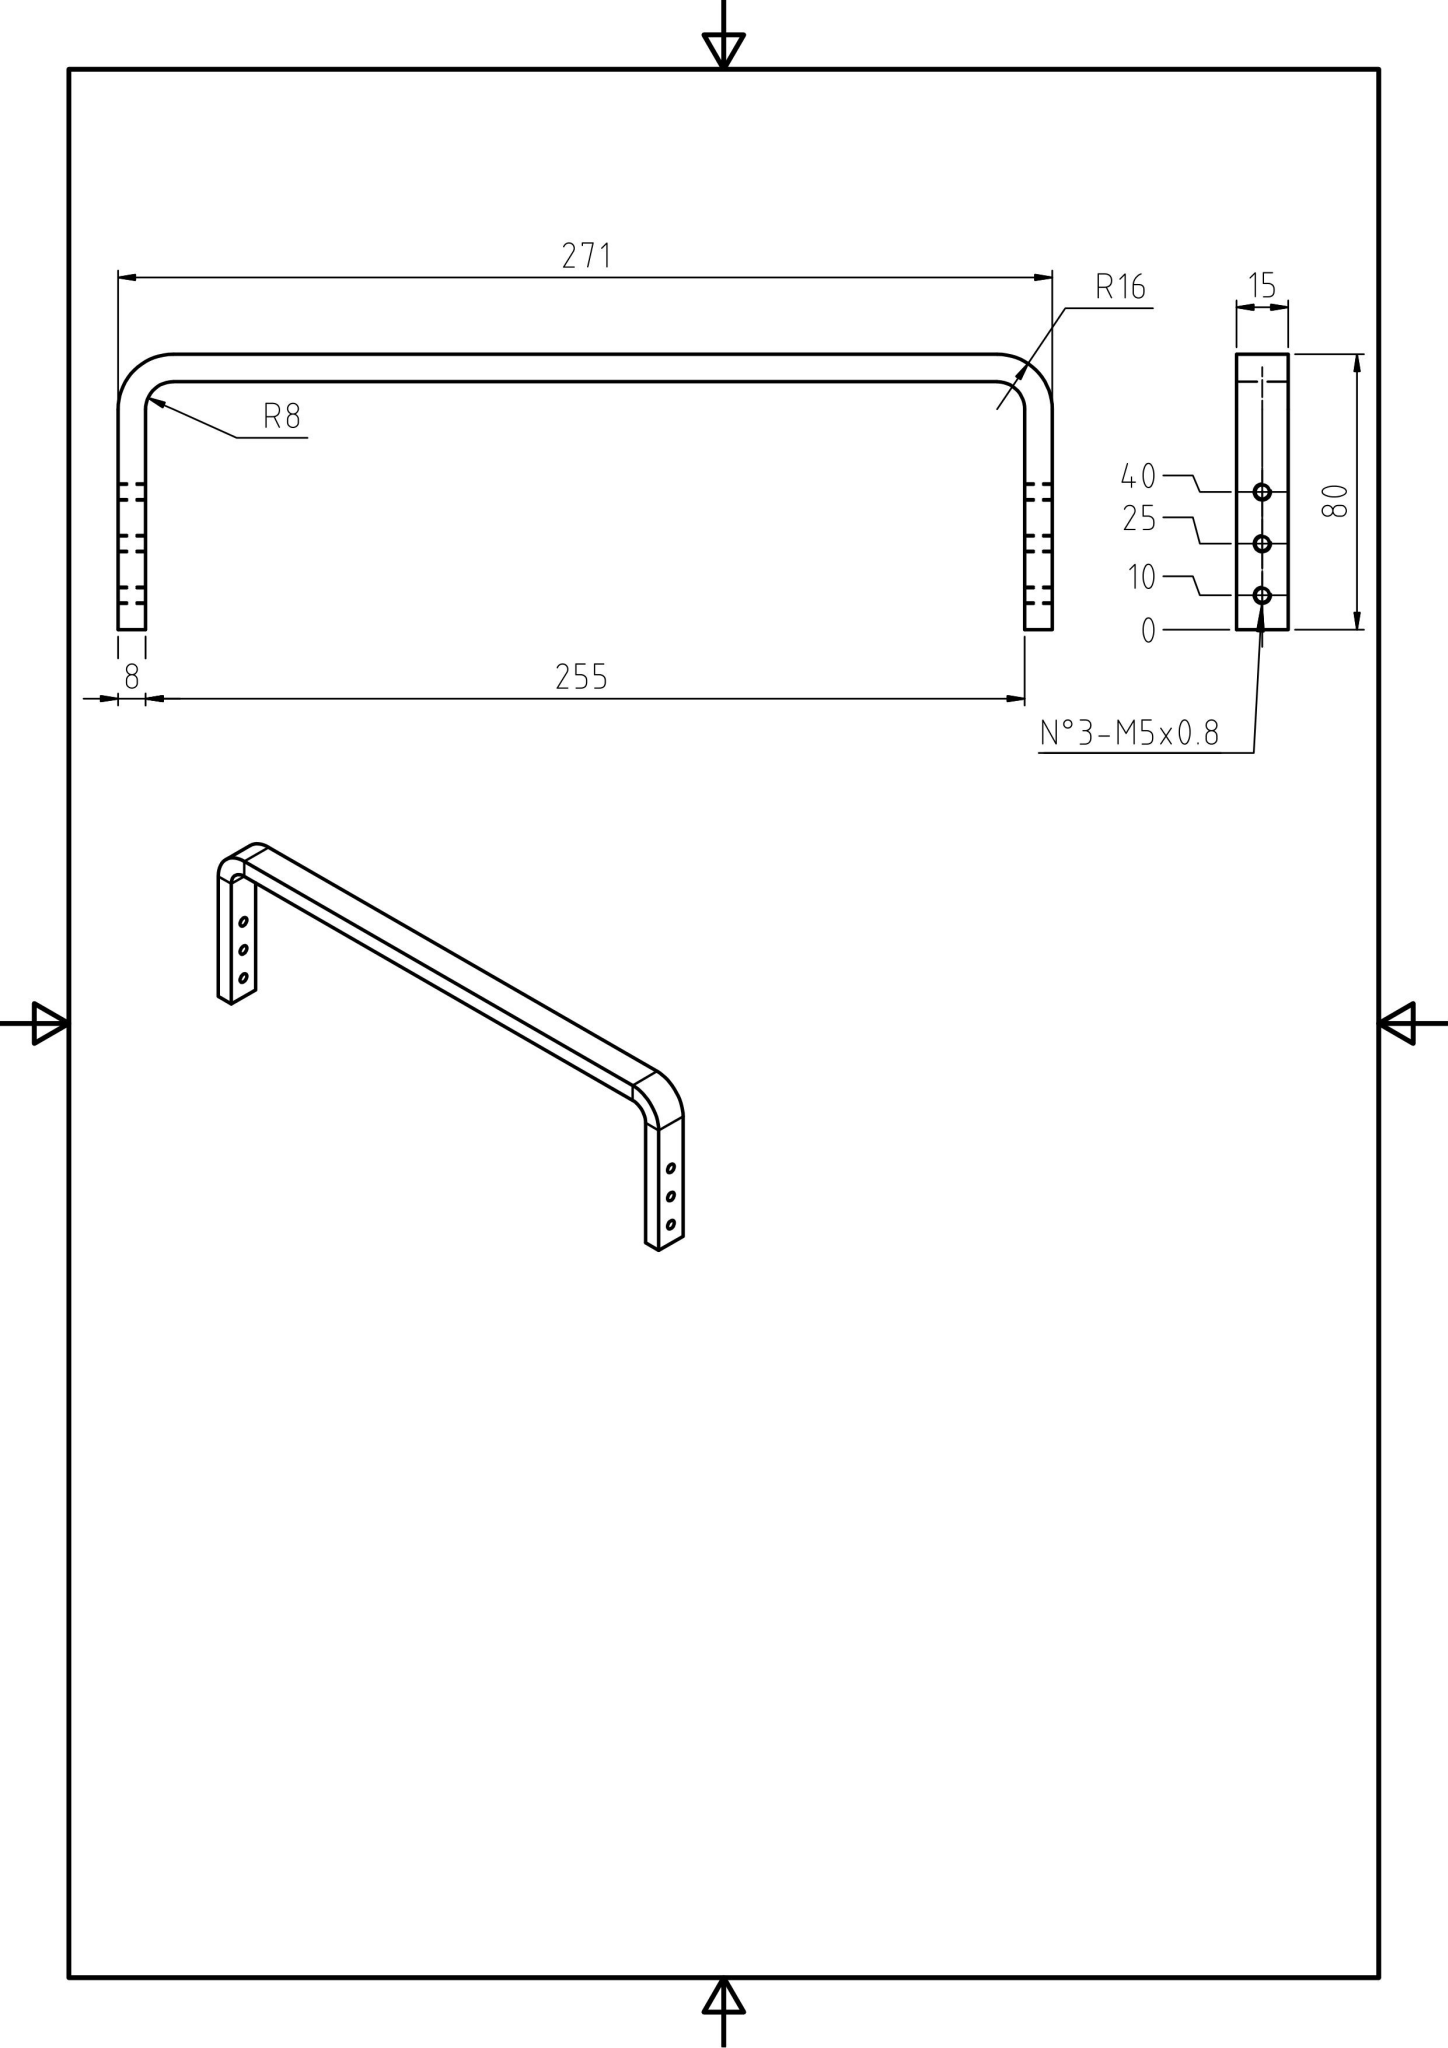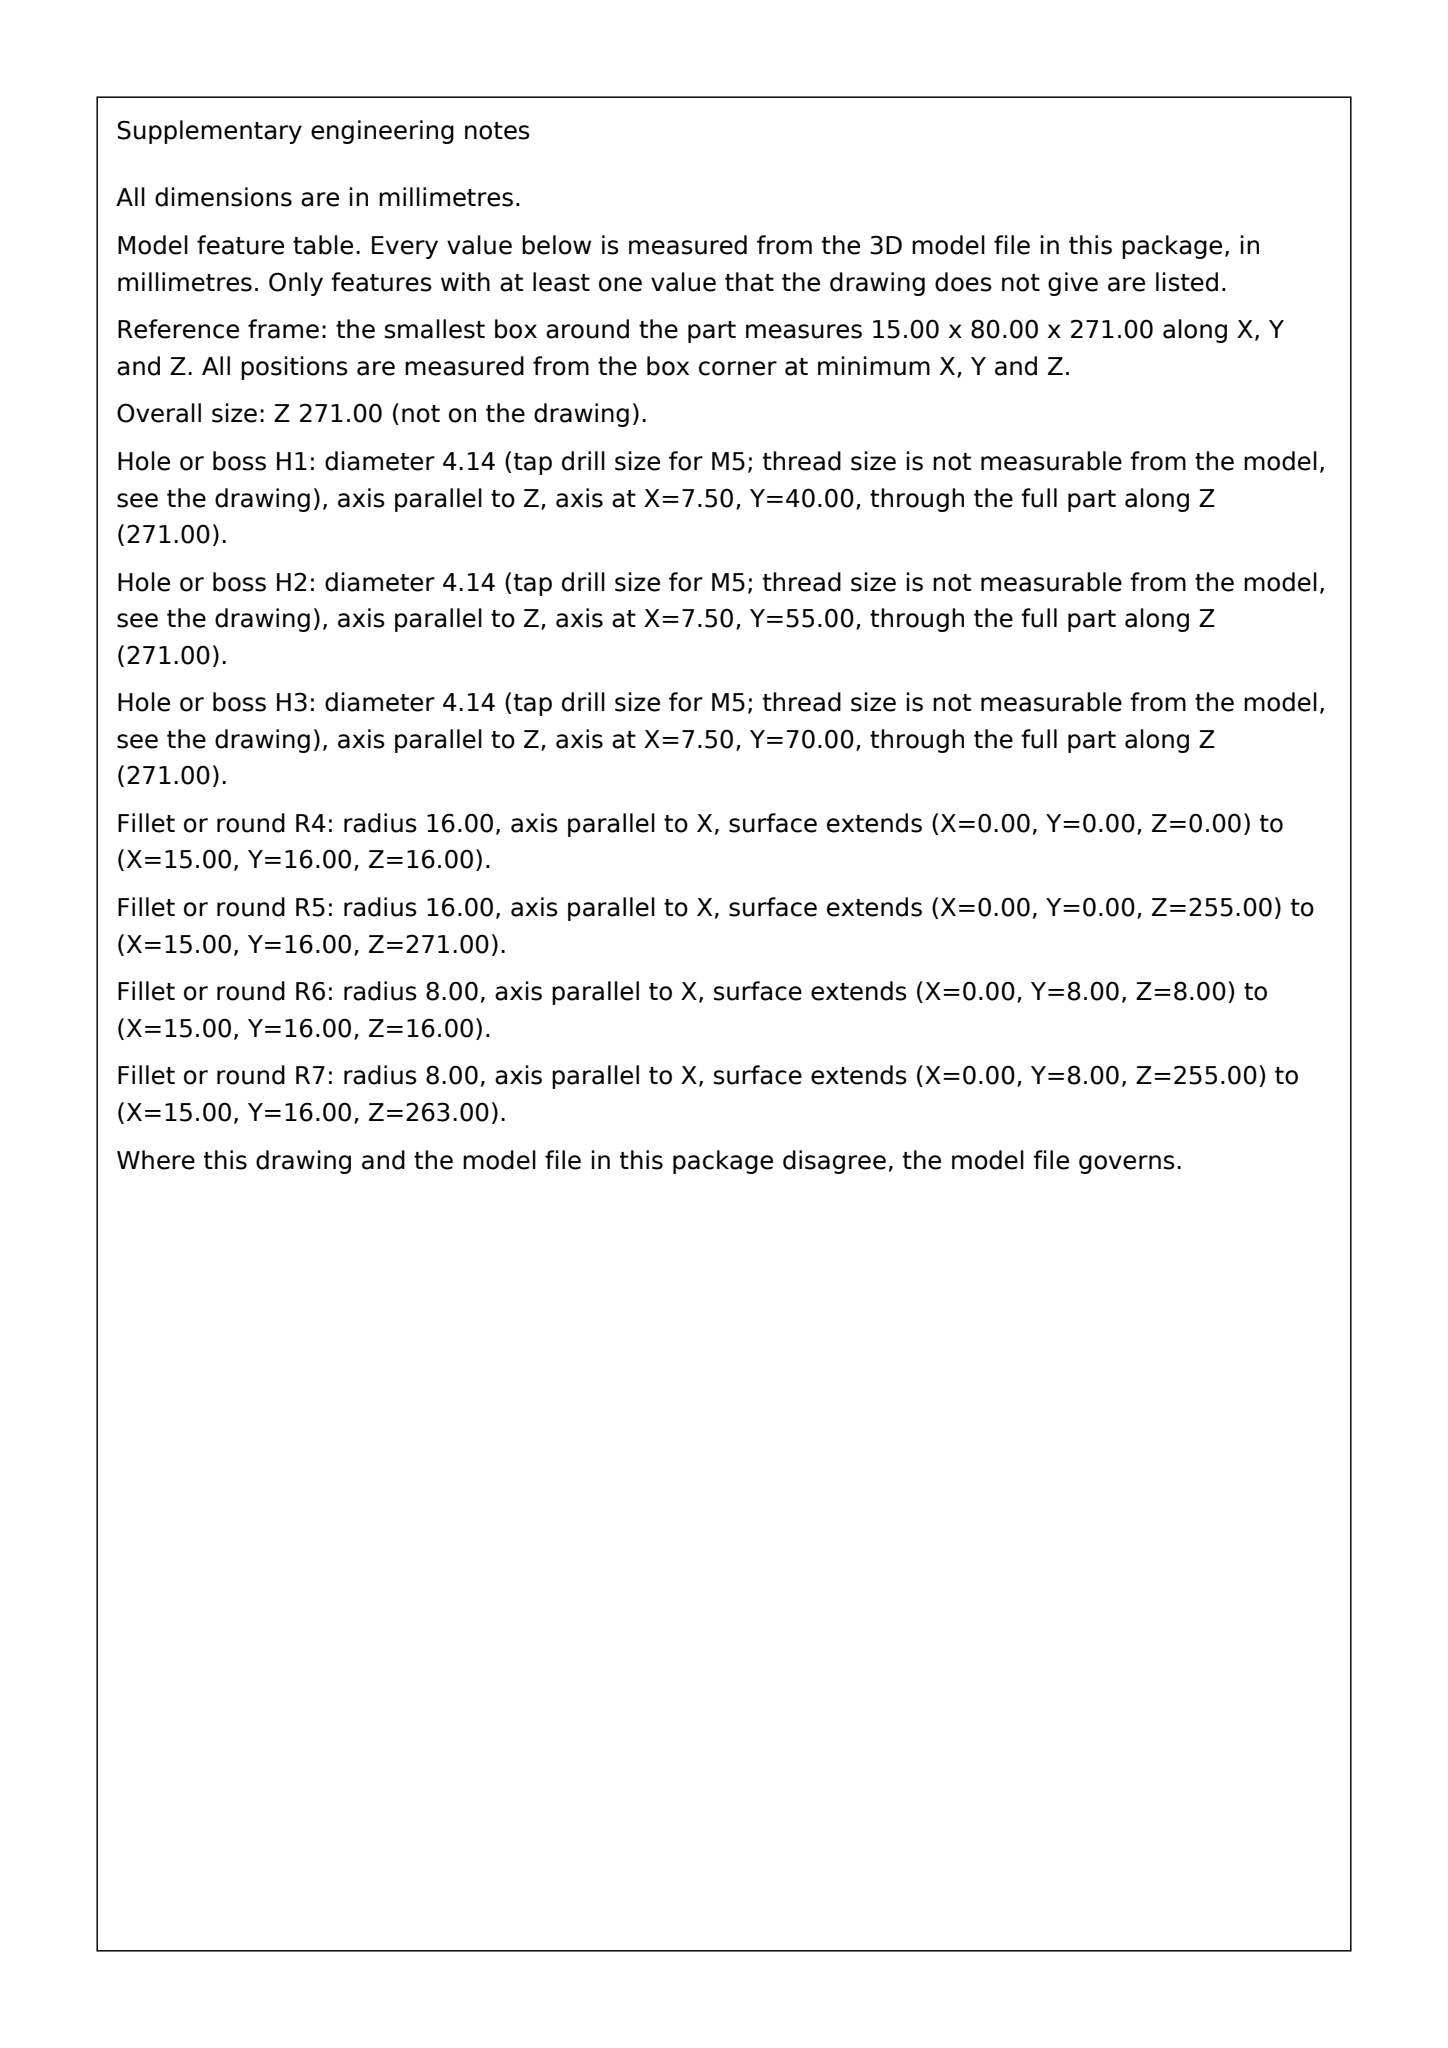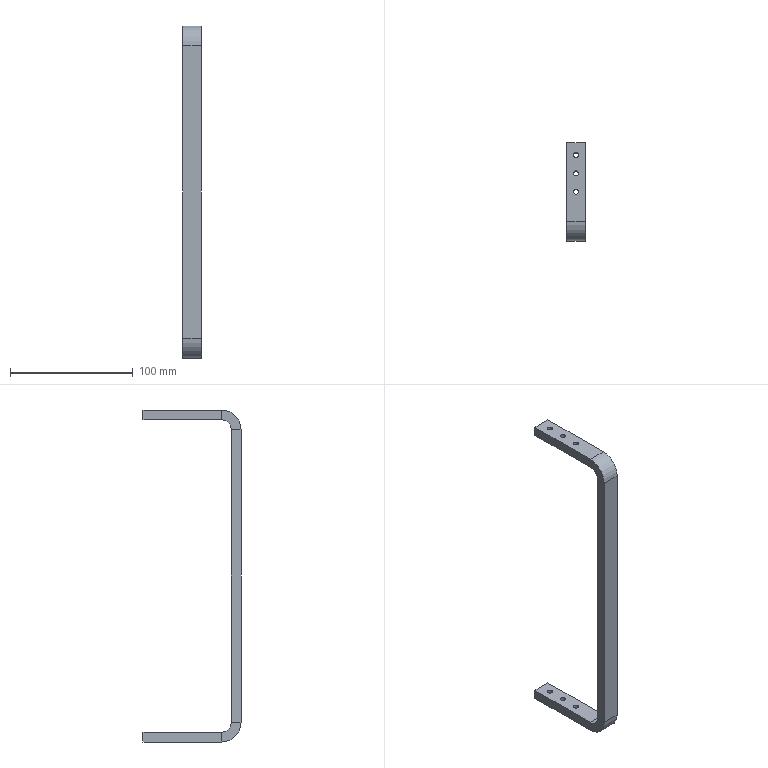Part | SolidWorks | mm | 1 solid | 34 faces | box 15 x 80 x 271 mm | volume 47920 mm3 | plane 18 | cylinder 16 | commonest cylinder face diameters 4.134 x12 32 x2 16 x2